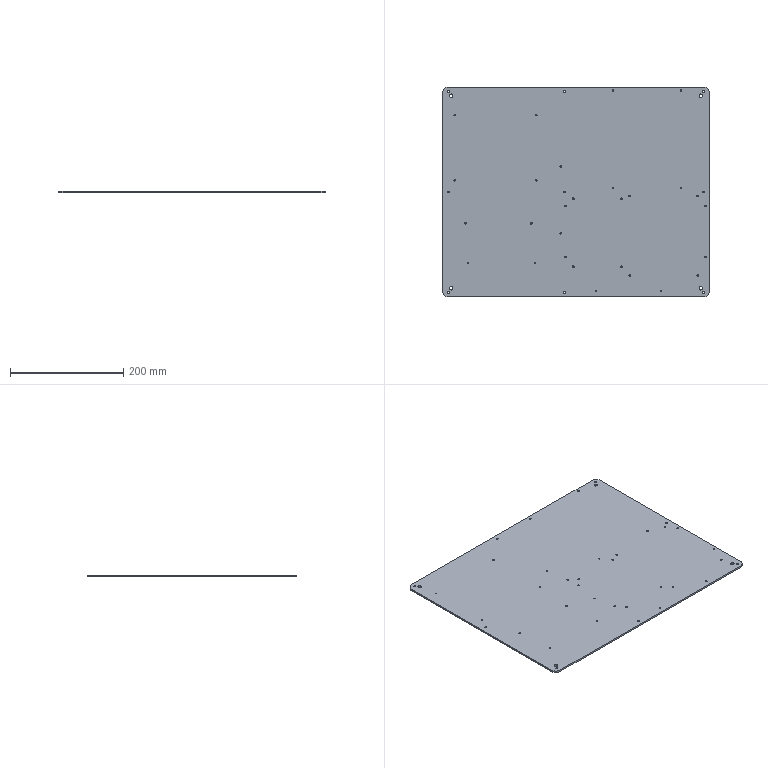CAM job | Mastercam | mm | 1 operations | part box 470 x 370 x 6
1. Drill/Counterbore | 7 - 4 倒角刀